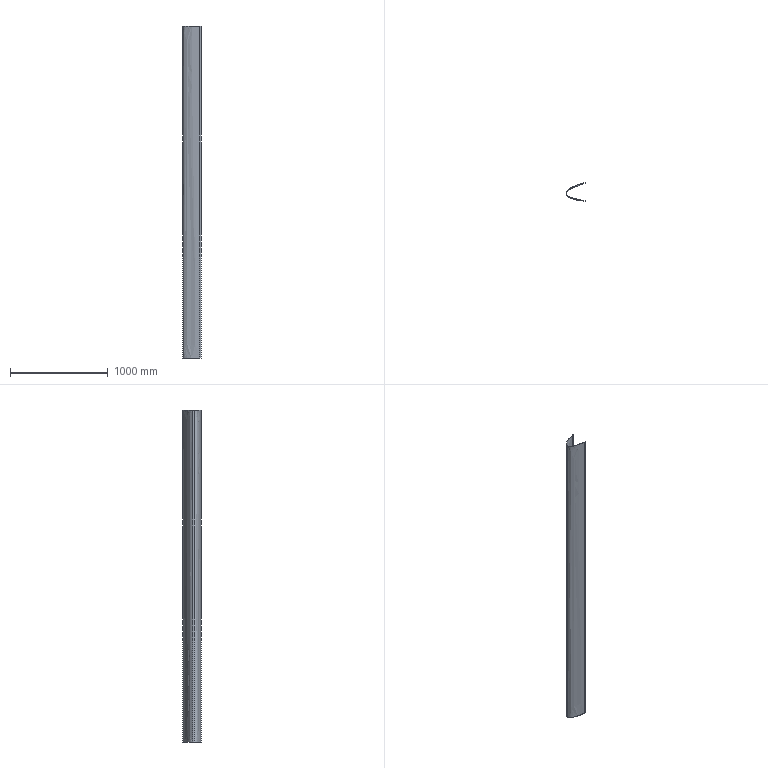Component | NX | SKIN_0_5_FRONT | 1 solid | 14 faces | volume 758573 mm3 | plane 8 | other 4 | cylinder 2 | commonest cylinder face diameters 97.613 x1 96.612 x1